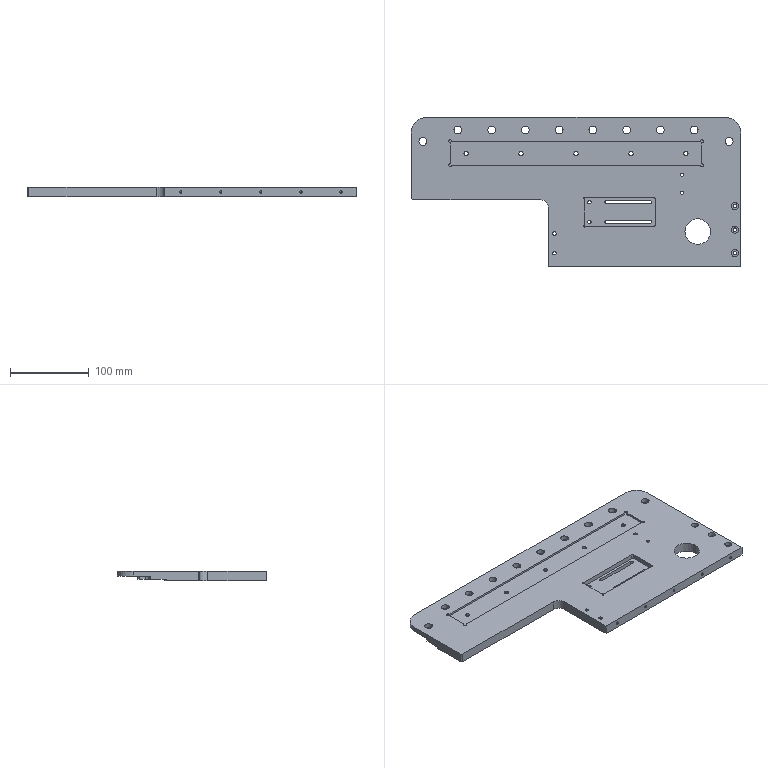Component | SolidWorks | 170423A4-PulleyRetainingPlate1-1 | 1 solid | 158 faces | box 420 x 190 x 12 mm | volume 613574 mm3 | cylinder 101 | plane 47 | cone 10 | commonest cylinder face diameters 10 x22 4.5 x20 3.3 x10 9 x10 11 x10 5.5 x10 4 x8 4.2 x4
build123d program:
from build123d import *

# Parameters (mm, degrees)
SKETCH1_W                                       = 420
SKETCH1_H                                       = 190
BOSS_EXTRUDE1_DEPTH                             = 6
F_10_0_10_DIAMETER_HOLE1_D                      = 10
FILLET2_R                                       = 20
SKETCH7_W                                       = 320.2
SKETCH7_H                                       = 30.5
CUT_EXTRUDE2_DEPTH                              = 2.5
F_10_0_10_DIAMETER_HOLE2_D                      = 10
BOSS_EXTRUDE2_DEPTH                             = 4
FILLET3_R                                       = 5
CHAMFER1_SIZE                                   = 2
SKETCH11_R                                      = 2
CUT_EXTRUDE3_DEPTH                              = 2.5
M5_HEX_SOCKET_HEAD_CAP_SCREW_CBORE1_D           = 5.5
M5_HEX_SOCKET_HEAD_CAP_SCREW_CBORE1_CBORE_D     = 11
M5_HEX_SOCKET_HEAD_CAP_SCREW_CBORE1_CBORE_DEPTH = 5
SKETCH15_W                                      = 420
SKETCH15_H                                      = 130
BOSS_EXTRUDE3_DEPTH                             = 2
SKETCH14_R                                      = 16.25
CUT_EXTRUDE4_DEPTH                              = 284.45
SKETCH17_W                                      = 90
SKETCH17_H                                      = 36.2
CUT_EXTRUDE5_DEPTH                              = 6
FILLET4_R                                       = 2
SKETCH18_R                                      = 1
CUT_EXTRUDE6_DEPTH                              = 6
SKETCH19_W                                      = 175
SKETCH19_H                                      = 85
CUT_EXTRUDE7_DEPTH                              = 284.45
FILLET5_R                                       = 10
CHAMFER2_SIZE                                   = 2
M5_TAPPED_HOLE1_D                               = 4.2
M4_HEX_SOCKET_HEAD_CAP_SCREW_CBORE1_D           = 4.5
M4_HEX_SOCKET_HEAD_CAP_SCREW_CBORE1_CBORE_D     = 9
M4_HEX_SOCKET_HEAD_CAP_SCREW_CBORE1_CBORE_DEPTH = 5
M4_HEX_SOCKET_HEAD_CAP_SCREW_CBORE2_D           = 4.5
M4_HEX_SOCKET_HEAD_CAP_SCREW_CBORE2_CBORE_D     = 9
M4_HEX_SOCKET_HEAD_CAP_SCREW_CBORE2_CBORE_DEPTH = 5
M4_TAPPED_HOLE1_D                               = 3.3
M4_TAPPED_HOLE1_DEPTH                           = 11.5
M4_TAPPED_HOLE1_TIP                             = 0.9914
F_4_5_4_5_DIAMETER_HOLE1_D                      = 4.5
CUT_EXTRUDE8_DEPTH                              = 284.45


with BuildPart() as part:
    # Sketch1 → Boss-Extrude1 (new body)
    with BuildSketch(Plane.XY):
        with Locations((0, 95)):
            Rectangle(SKETCH1_W, SKETCH1_H)
    extrude(amount=BOSS_EXTRUDE1_DEPTH)

    # 10.0 _10_ Diameter Hole1 (through all)
    with Locations(Plane.XY.offset(6)):
        with Locations((-195, 159.5), (195, 159.5)):
            Hole(F_10_0_10_DIAMETER_HOLE1_D / 2)

    # Fillet2
    fillet2_edges = [part.edges().sort_by_distance(p)[0] for p in [
        (-210, 190, 3),
        (210, 190, 3),
    ]]
    fillet(fillet2_edges, radius=FILLET2_R)

    # Sketch7 → Cut-Extrude2 (cut)
    with BuildSketch(Plane.XY.offset(6)):
        with Locations((0, 144.25)):
            Rectangle(SKETCH7_W, SKETCH7_H)
    extrude(amount=-CUT_EXTRUDE2_DEPTH, mode=Mode.SUBTRACT)

    # 10.0 _10_ Diameter Hole2 (through all)
    with Locations(Plane.XY.offset(6)):
        with Locations((-150.5, 174), (-107.5, 174), (-64.5, 174), (-21.5, 174), (21.5, 174), (64.5, 174), (107.5, 174), (150.5, 174)):
            Hole(F_10_0_10_DIAMETER_HOLE2_D / 2)

    # Sketch10 → Boss-Extrude2 (add)
    with BuildSketch(Plane(origin=(0, 0, 0), x_dir=(-1, 0, 0), z_dir=(0, 0, -1))):
        Polygon((-210, 0), (-210, 149.5), (-185, 149.5), (-185, 164), (185, 164), (185, 149.5), (210, 149.5), (210, 0), align=None)
    extrude(amount=BOSS_EXTRUDE2_DEPTH)

    # Fillet3
    fillet3_edges = [part.edges().sort_by_distance(p)[0] for p in [
        (-185, 149.5, -2),
        (185, 149.5, -2),
    ]]
    fillet(fillet3_edges, radius=FILLET3_R)

    # Chamfer1
    chamfer1_edges = [part.edges().sort_by_distance(p)[0] for p in [
        (-210, 149.5, -2),
        (-185, 164, -2),
        (185, 164, -2),
        (210, 149.5, -2),
    ]]
    chamfer(chamfer1_edges, length=CHAMFER1_SIZE)

    # Sketch11 → Cut-Extrude3 (cut)
    with BuildSketch(Plane.XY.offset(6)):
        with Locations((-160.1, 129)):
            Circle(SKETCH11_R)
        with Locations((-160.1, 159.5)):
            Circle(SKETCH11_R)
        with Locations((160.1, 159.5)):
            Circle(SKETCH11_R)
        with Locations((160.1, 129)):
            Circle(SKETCH11_R)
    extrude(amount=-CUT_EXTRUDE3_DEPTH, mode=Mode.SUBTRACT)

    # M5 Hex Socket Head Cap Screw CBORE1 (through all)
    with Locations(Plane(origin=(0, 0, -4), x_dir=(-1, 0, 0), z_dir=(0, 0, -1))):
        with Locations((140, 144), (-140, 144), (-70, 144), (0, 144), (70, 144)):
            CounterBoreHole(M5_HEX_SOCKET_HEAD_CAP_SCREW_CBORE1_D / 2, M5_HEX_SOCKET_HEAD_CAP_SCREW_CBORE1_CBORE_D / 2, M5_HEX_SOCKET_HEAD_CAP_SCREW_CBORE1_CBORE_DEPTH)

    # Sketch15 → Boss-Extrude3 (add)
    with BuildSketch(Plane(origin=(0, 0, -4), x_dir=(-1, 0, 0), z_dir=(0, 0, -1))):
        with Locations((0, 65)):
            Rectangle(SKETCH15_W, SKETCH15_H)
    extrude(amount=BOSS_EXTRUDE3_DEPTH)

    # Sketch14 → Cut-Extrude4 (cut, through all)
    with BuildSketch(Plane(origin=(0, 0, -6), x_dir=(-1, 0, 0), z_dir=(0, 0, -1))):
        with Locations((-155, 44.5)):
            Circle(SKETCH14_R)
    extrude(amount=-CUT_EXTRUDE4_DEPTH, mode=Mode.SUBTRACT)

    # Sketch17 → Cut-Extrude5 (cut)
    with BuildSketch(Plane.XY.offset(6)):
        with Locations((56, 69.5)):
            Rectangle(SKETCH17_W, SKETCH17_H)
    extrude(amount=-CUT_EXTRUDE5_DEPTH, mode=Mode.SUBTRACT)

    # Fillet4
    fillet4_edges = [part.edges().sort_by_distance(p)[0] for p in [
        (101, 87.6, 3),
        (101, 51.4, 3),
    ]]
    fillet(fillet4_edges, radius=FILLET4_R)

    # Sketch18 → Cut-Extrude6 (cut)
    with BuildSketch(Plane.XY.offset(6)):
        with Locations((11, 87.6)):
            Circle(SKETCH18_R)
        with Locations((11, 51.4)):
            Circle(SKETCH18_R)
    extrude(amount=-CUT_EXTRUDE6_DEPTH, mode=Mode.SUBTRACT)

    # Sketch19 → Cut-Extrude7 (cut, through all)
    with BuildSketch(Plane.XY.offset(6)):
        with Locations((-122.5, 42.5)):
            Rectangle(SKETCH19_W, SKETCH19_H)
    extrude(amount=-CUT_EXTRUDE7_DEPTH, mode=Mode.SUBTRACT)

    # Fillet5
    fillet5_edges = [part.edges().sort_by_distance(p)[0] for p in [
        (-35, 85, 0),
    ]]
    fillet(fillet5_edges, radius=FILLET5_R)

    # Chamfer2
    chamfer2_edges = [part.edges().sort_by_distance(p)[0] for p in [
        (210, 130, -5),
        (-210, 130, -5),
        (-210, 85, 0),
    ]]
    chamfer(chamfer2_edges, length=CHAMFER2_SIZE)

    # M5 Tapped Hole1 (through all)
    with Locations(Plane.XY.offset(6)):
        with Locations((135, 117), (135, 94)):
            Hole(M5_TAPPED_HOLE1_D / 2)

    # M4 Hex Socket Head Cap Screw CBORE1 (through all)
    with Locations(Plane.XY.offset(6)):
        with Locations((202.5, 77), (202.5, 47), (202.5, 17)):
            CounterBoreHole(M4_HEX_SOCKET_HEAD_CAP_SCREW_CBORE1_D / 2, M4_HEX_SOCKET_HEAD_CAP_SCREW_CBORE1_CBORE_D / 2, M4_HEX_SOCKET_HEAD_CAP_SCREW_CBORE1_CBORE_DEPTH)

    # M4 Hex Socket Head Cap Screw CBORE2 (through all)
    with Locations(Plane(origin=(0, 0, -6), x_dir=(-1, 0, 0), z_dir=(0, 0, -1))):
        with Locations((27.5, 42), (27.5, 17)):
            CounterBoreHole(M4_HEX_SOCKET_HEAD_CAP_SCREW_CBORE2_D / 2, M4_HEX_SOCKET_HEAD_CAP_SCREW_CBORE2_CBORE_D / 2, M4_HEX_SOCKET_HEAD_CAP_SCREW_CBORE2_CBORE_DEPTH)

    # M4 Tapped Hole1
    with Locations(Plane(origin=(0, 0, 0), x_dir=(-1, 0, 0), z_dir=(0, -1, 0))):
        with Locations((14.5, 0), (-189.5, 0), (-138.5, 0), (-87.5, 0), (-36.5, 0)):
            Hole(M4_TAPPED_HOLE1_D / 2, depth=M4_TAPPED_HOLE1_DEPTH)
            with Locations((0, 0, -(M4_TAPPED_HOLE1_DEPTH + M4_TAPPED_HOLE1_TIP / 2))):  # 118° drill point
                Cone(0, M4_TAPPED_HOLE1_D / 2, M4_TAPPED_HOLE1_TIP, mode=Mode.SUBTRACT)

    # 4.5 _4.5_ Diameter Hole1 (through all)
    with Locations(Plane(origin=(0, 0, -6), x_dir=(-1, 0, 0), z_dir=(0, 0, -1))):
        with Locations((-17, 57), (-17, 82)):
            Hole(F_4_5_4_5_DIAMETER_HOLE1_D / 2)

    # Sketch30 → Cut-Extrude8 (cut, through all)
    with BuildSketch(Plane(origin=(0, 0, -6), x_dir=(-1, 0, 0), z_dir=(0, 0, -1))):
        with BuildLine():
            Line((-94, 84.25), (-39, 84.25))
            ThreePointArc((-39, 84.25), (-36.75, 82), (-39, 79.75))
            Line((-39, 79.75), (-94, 79.75))
            ThreePointArc((-94, 79.75), (-96.25, 82), (-94, 84.25))
        make_face()
        with BuildLine():
            Line((-94, 59.25), (-39, 59.25))
            ThreePointArc((-39, 59.25), (-36.75, 57), (-39, 54.75))
            Line((-39, 54.75), (-94, 54.75))
            ThreePointArc((-94, 54.75), (-96.25, 57), (-94, 59.25))
        make_face()
    extrude(amount=-CUT_EXTRUDE8_DEPTH, mode=Mode.SUBTRACT)


solid = part.part

# Placed as in the assembly
solid = solid.moved(Location((-55.246, -165.288, 415), (0, 0, 0)))